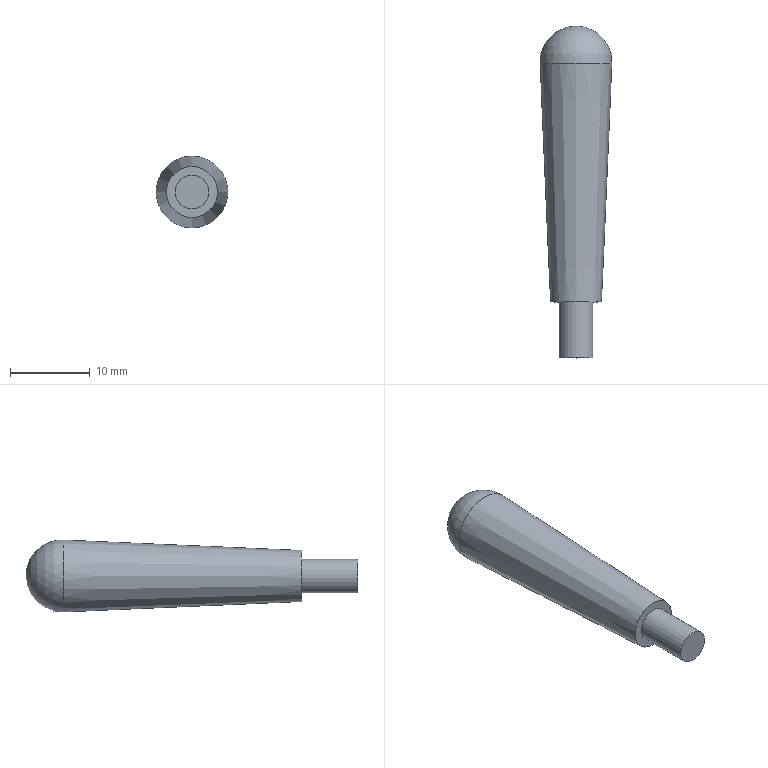Component | NX | HANDLE | 1 solid | 5 faces | box 9 x 41.5 x 9 mm | volume 1698 mm3 | plane 2 | sphere 1 | cone 1 | cylinder 1 | commonest cylinder face diameters 4.2 x1
STEP:
#1=CARTESIAN_POINT('',(0.,0.,0.));
#2=DIRECTION('',(0.,0.,1.));
#3=DIRECTION('',(1.,0.,0.));
#4=AXIS2_PLACEMENT_3D('',#1,#2,#3);
#5=CARTESIAN_POINT('',(0.,69.,123.5));
#6=VERTEX_POINT('',#5);
#7=CARTESIAN_POINT('',(0.,69.,125.6));
#8=DIRECTION('',(0.,-1.,0.));
#9=DIRECTION('',(0.,0.,-1.));
#10=AXIS2_PLACEMENT_3D('',#7,#8,#9);
#11=CIRCLE('',#10,2.1);
#12=CARTESIAN_POINT('',(0.,69.,127.7));
#13=DIRECTION('',(0.,1.,0.));
#14=DIRECTION('',(0.,0.,1.));
#15=AXIS2_PLACEMENT_3D('',#12,#13,#14);
#16=PLANE('',#15);
#17=CARTESIAN_POINT('',(-4.2,0.));
#18=CARTESIAN_POINT('',(-4.2,3.637));
#19=CARTESIAN_POINT('',(-1.05,1.819));
#20=CARTESIAN_POINT('',(2.1,0.));
#21=CARTESIAN_POINT('',(-1.05,-1.819));
#22=CARTESIAN_POINT('',(-4.2,-3.637));
#23=CARTESIAN_POINT('',(-4.2,0.));
#24=(BOUNDED_CURVE()B_SPLINE_CURVE(2,(#17,#18,#19,#20,#21,#22,#23),.UNSPECIFIED.,.T.,.F.)B_SPLINE_CURVE_WITH_KNOTS((1,2,2,2,2,1),(-2.094,0.,2.094,4.189,6.283,8.378),.UNSPECIFIED.)CURVE()GEOMETRIC_REPRESENTATION_ITEM()RATIONAL_B_SPLINE_CURVE((1.,0.5,1.,0.5,1.,0.5,1.))REPRESENTATION_ITEM(''));
#25=(GEOMETRIC_REPRESENTATION_CONTEXT(2)PARAMETRIC_REPRESENTATION_CONTEXT()REPRESENTATION_CONTEXT('',''));
#26=DEFINITIONAL_REPRESENTATION('',(#24),#25);
#27=PCURVE('',#16,#26);
#28=CARTESIAN_POINT('',(0.,69.,125.6));
#29=DIRECTION('',(0.,-1.,0.));
#30=DIRECTION('',(0.,0.,-1.));
#31=AXIS2_PLACEMENT_3D('',#28,#29,#30);
#32=CYLINDRICAL_SURFACE('',#31,2.1);
#33=CARTESIAN_POINT('',(0.,0.));
#34=DIRECTION('',(1.,0.));
#35=VECTOR('',#34,1.);
#36=LINE('',#33,#35);
#37=(GEOMETRIC_REPRESENTATION_CONTEXT(2)PARAMETRIC_REPRESENTATION_CONTEXT()REPRESENTATION_CONTEXT('',''));
#38=DEFINITIONAL_REPRESENTATION('',(#36),#37);
#39=PCURVE('',#32,#38);
#40=SURFACE_CURVE('',#11,(#27,#39),.PCURVE_S1.);
#41=EDGE_CURVE('',#6,#6,#40,.T.);
#42=ORIENTED_EDGE('',*,*,#41,.T.);
#43=EDGE_LOOP('',(#42));
#44=FACE_BOUND('',#43,.T.);
#45=ADVANCED_FACE('',(#44),#16,.F.);
#46=CARTESIAN_POINT('',(-0.,105.804,130.096));
#47=VERTEX_POINT('',#46);
#48=CARTESIAN_POINT('',(0.,105.804,121.104));
#49=VERTEX_POINT('',#48);
#50=CARTESIAN_POINT('',(0.,105.804,125.6));
#51=DIRECTION('',(0.,-1.,0.));
#52=DIRECTION('',(0.,0.,-1.));
#53=AXIS2_PLACEMENT_3D('',#50,#51,#52);
#54=CIRCLE('',#53,4.496);
#55=CARTESIAN_POINT('',(0.,106.,125.6));
#56=DIRECTION('',(0.,-1.,0.));
#57=DIRECTION('',(0.,0.,1.));
#58=AXIS2_PLACEMENT_3D('',#55,#56,#57);
#59=SPHERICAL_SURFACE('',#58,4.5);
#60=CARTESIAN_POINT('',(-3.142,0.04363));
#61=CARTESIAN_POINT('',(-3.046,0.04363));
#62=CARTESIAN_POINT('',(-2.856,0.04363));
#63=CARTESIAN_POINT('',(-2.57,0.04363));
#64=CARTESIAN_POINT('',(-2.285,0.04363));
#65=CARTESIAN_POINT('',(-1.999,0.04363));
#66=CARTESIAN_POINT('',(-1.714,0.04363));
#67=CARTESIAN_POINT('',(-1.428,0.04363));
#68=CARTESIAN_POINT('',(-1.142,0.04363));
#69=CARTESIAN_POINT('',(-0.8568,0.04363));
#70=CARTESIAN_POINT('',(-0.5712,0.04363));
#71=CARTESIAN_POINT('',(-0.2856,0.04363));
#72=CARTESIAN_POINT('',(0.,0.04363));
#73=CARTESIAN_POINT('',(0.2856,0.04363));
#74=CARTESIAN_POINT('',(0.5712,0.04363));
#75=CARTESIAN_POINT('',(0.8568,0.04363));
#76=CARTESIAN_POINT('',(1.142,0.04363));
#77=CARTESIAN_POINT('',(1.428,0.04363));
#78=CARTESIAN_POINT('',(1.714,0.04363));
#79=CARTESIAN_POINT('',(1.999,0.04363));
#80=CARTESIAN_POINT('',(2.285,0.04363));
#81=CARTESIAN_POINT('',(2.57,0.04363));
#82=CARTESIAN_POINT('',(2.856,0.04363));
#83=CARTESIAN_POINT('',(3.046,0.04363));
#84=CARTESIAN_POINT('',(3.142,0.04363));
#85=B_SPLINE_CURVE_WITH_KNOTS('',3,(#60,#61,#62,#63,#64,#65,#66,#67,#68,#69,#70,#71,#72,#73,#74,#75,#76,#77,#78,#79,#80,#81,#82,#83,#84),.UNSPECIFIED.,.F.,.F.,(4,1,1,1,1,1,1,1,1,1,1,1,1,1,1,1,1,1,1,1,1,1,4),(0.,0.2856,0.5712,0.8568,1.142,1.428,1.714,1.999,2.285,2.57,2.856,3.142,3.427,3.713,3.998,4.284,4.57,4.855,5.141,5.426,5.712,5.998,6.283),.QUASI_UNIFORM_KNOTS.);
#86=(GEOMETRIC_REPRESENTATION_CONTEXT(2)PARAMETRIC_REPRESENTATION_CONTEXT()REPRESENTATION_CONTEXT('',''));
#87=DEFINITIONAL_REPRESENTATION('',(#85),#86);
#88=PCURVE('',#59,#87);
#89=CARTESIAN_POINT('',(0.,105.804,125.6));
#90=DIRECTION('',(0.,1.,0.));
#91=DIRECTION('',(0.,0.,1.));
#92=AXIS2_PLACEMENT_3D('',#89,#90,#91);
#93=CONICAL_SURFACE('',#92,4.496,0.04363);
#94=CARTESIAN_POINT('',(9.425,0.));
#95=DIRECTION('',(-1.,0.));
#96=VECTOR('',#95,1.);
#97=LINE('',#94,#96);
#98=(GEOMETRIC_REPRESENTATION_CONTEXT(2)PARAMETRIC_REPRESENTATION_CONTEXT()REPRESENTATION_CONTEXT('',''));
#99=DEFINITIONAL_REPRESENTATION('',(#97),#98);
#100=PCURVE('',#93,#99);
#101=SURFACE_CURVE('',#54,(#88,#100),.PCURVE_S1.);
#102=EDGE_CURVE('',#47,#49,#101,.T.);
#103=ORIENTED_EDGE('',*,*,#102,.F.);
#104=CARTESIAN_POINT('',(0.,110.5,125.6));
#105=VERTEX_POINT('',#104);
#106=CARTESIAN_POINT('',(-0.,110.5,125.6));
#107=CARTESIAN_POINT('',(0.,110.5,126.811));
#108=CARTESIAN_POINT('',(0.,110.109,128.022));
#109=CARTESIAN_POINT('',(0.,109.327,129.075));
#110=CARTESIAN_POINT('',(0.,108.24,129.811));
#111=CARTESIAN_POINT('',(0.,107.013,130.149));
#112=CARTESIAN_POINT('',(0.,105.804,130.096));
#113=B_SPLINE_CURVE_WITH_KNOTS('',6,(#106,#107,#108,#109,#110,#111,#112),.UNSPECIFIED.,.F.,.F.,(7,7),(-1.571,0.04363),.PIECEWISE_BEZIER_KNOTS.);
#114=CARTESIAN_POINT('',(0.,0.));
#115=DIRECTION('',(0.,1.));
#116=VECTOR('',#115,1.);
#117=LINE('',#114,#116);
#118=(GEOMETRIC_REPRESENTATION_CONTEXT(2)PARAMETRIC_REPRESENTATION_CONTEXT()REPRESENTATION_CONTEXT('',''));
#119=DEFINITIONAL_REPRESENTATION('',(#117),#118);
#120=PCURVE('',#59,#119);
#121=CARTESIAN_POINT('',(6.283,0.));
#122=DIRECTION('',(0.,1.));
#123=VECTOR('',#122,1.);
#124=LINE('',#121,#123);
#125=(GEOMETRIC_REPRESENTATION_CONTEXT(2)PARAMETRIC_REPRESENTATION_CONTEXT()REPRESENTATION_CONTEXT('',''));
#126=DEFINITIONAL_REPRESENTATION('',(#124),#125);
#127=PCURVE('',#59,#126);
#128=SEAM_CURVE('',#113,(#120,#127),.PCURVE_S1.);
#129=EDGE_CURVE('',#105,#47,#128,.T.);
#130=ORIENTED_EDGE('',*,*,#129,.F.);
#131=ORIENTED_EDGE('',*,*,#129,.T.);
#132=CARTESIAN_POINT('',(0.,105.804,125.6));
#133=DIRECTION('',(0.,-1.,0.));
#134=DIRECTION('',(0.,0.,-1.));
#135=AXIS2_PLACEMENT_3D('',#132,#133,#134);
#136=CIRCLE('',#135,4.496);
#137=CARTESIAN_POINT('',(3.142,0.04363));
#138=CARTESIAN_POINT('',(3.237,0.04363));
#139=CARTESIAN_POINT('',(3.427,0.04363));
#140=CARTESIAN_POINT('',(3.713,0.04363));
#141=CARTESIAN_POINT('',(3.998,0.04363));
#142=CARTESIAN_POINT('',(4.284,0.04363));
#143=CARTESIAN_POINT('',(4.57,0.04363));
#144=CARTESIAN_POINT('',(4.855,0.04363));
#145=CARTESIAN_POINT('',(5.141,0.04363));
#146=CARTESIAN_POINT('',(5.426,0.04363));
#147=CARTESIAN_POINT('',(5.712,0.04363));
#148=CARTESIAN_POINT('',(5.998,0.04363));
#149=CARTESIAN_POINT('',(6.283,0.04363));
#150=CARTESIAN_POINT('',(6.569,0.04363));
#151=CARTESIAN_POINT('',(6.854,0.04363));
#152=CARTESIAN_POINT('',(7.14,0.04363));
#153=CARTESIAN_POINT('',(7.426,0.04363));
#154=CARTESIAN_POINT('',(7.711,0.04363));
#155=CARTESIAN_POINT('',(7.997,0.04363));
#156=CARTESIAN_POINT('',(8.282,0.04363));
#157=CARTESIAN_POINT('',(8.568,0.04363));
#158=CARTESIAN_POINT('',(8.854,0.04363));
#159=CARTESIAN_POINT('',(9.139,0.04363));
#160=CARTESIAN_POINT('',(9.33,0.04363));
#161=CARTESIAN_POINT('',(9.425,0.04363));
#162=B_SPLINE_CURVE_WITH_KNOTS('',3,(#137,#138,#139,#140,#141,#142,#143,#144,#145,#146,#147,#148,#149,#150,#151,#152,#153,#154,#155,#156,#157,#158,#159,#160,#161),.UNSPECIFIED.,.F.,.F.,(4,1,1,1,1,1,1,1,1,1,1,1,1,1,1,1,1,1,1,1,1,1,4),(0.,0.2856,0.5712,0.8568,1.142,1.428,1.714,1.999,2.285,2.57,2.856,3.142,3.427,3.713,3.998,4.284,4.57,4.855,5.141,5.426,5.712,5.998,6.283),.QUASI_UNIFORM_KNOTS.);
#163=(GEOMETRIC_REPRESENTATION_CONTEXT(2)PARAMETRIC_REPRESENTATION_CONTEXT()REPRESENTATION_CONTEXT('',''));
#164=DEFINITIONAL_REPRESENTATION('',(#162),#163);
#165=PCURVE('',#59,#164);
#166=CARTESIAN_POINT('',(9.425,0.));
#167=DIRECTION('',(-1.,0.));
#168=VECTOR('',#167,1.);
#169=LINE('',#166,#168);
#170=(GEOMETRIC_REPRESENTATION_CONTEXT(2)PARAMETRIC_REPRESENTATION_CONTEXT()REPRESENTATION_CONTEXT('',''));
#171=DEFINITIONAL_REPRESENTATION('',(#169),#170);
#172=PCURVE('',#93,#171);
#173=SURFACE_CURVE('',#136,(#165,#172),.PCURVE_S1.);
#174=EDGE_CURVE('',#49,#47,#173,.T.);
#175=ORIENTED_EDGE('',*,*,#174,.F.);
#176=EDGE_LOOP('',(#103,#130,#131,#175));
#177=FACE_BOUND('',#176,.T.);
#178=ADVANCED_FACE('',(#177),#59,.T.);
#179=CARTESIAN_POINT('',(0.,76.,122.406));
#180=VERTEX_POINT('',#179);
#181=CARTESIAN_POINT('',(0.,76.,125.6));
#182=DIRECTION('',(0.,-1.,0.));
#183=DIRECTION('',(0.,0.,-1.));
#184=AXIS2_PLACEMENT_3D('',#181,#182,#183);
#185=CIRCLE('',#184,3.194);
#186=CARTESIAN_POINT('',(9.425,-29.804));
#187=DIRECTION('',(-1.,0.));
#188=VECTOR('',#187,1.);
#189=LINE('',#186,#188);
#190=(GEOMETRIC_REPRESENTATION_CONTEXT(2)PARAMETRIC_REPRESENTATION_CONTEXT()REPRESENTATION_CONTEXT('',''));
#191=DEFINITIONAL_REPRESENTATION('',(#189),#190);
#192=PCURVE('',#93,#191);
#193=CARTESIAN_POINT('',(0.,76.,128.794));
#194=DIRECTION('',(0.,1.,0.));
#195=DIRECTION('',(0.,0.,1.));
#196=AXIS2_PLACEMENT_3D('',#193,#194,#195);
#197=PLANE('',#196);
#198=CARTESIAN_POINT('',(-6.389,0.));
#199=CARTESIAN_POINT('',(-6.389,5.533));
#200=CARTESIAN_POINT('',(-1.597,2.766));
#201=CARTESIAN_POINT('',(3.194,0.));
#202=CARTESIAN_POINT('',(-1.597,-2.766));
#203=CARTESIAN_POINT('',(-6.389,-5.533));
#204=CARTESIAN_POINT('',(-6.389,0.));
#205=(BOUNDED_CURVE()B_SPLINE_CURVE(2,(#198,#199,#200,#201,#202,#203,#204),.UNSPECIFIED.,.T.,.F.)B_SPLINE_CURVE_WITH_KNOTS((1,2,2,2,2,1),(-2.094,0.,2.094,4.189,6.283,8.378),.UNSPECIFIED.)CURVE()GEOMETRIC_REPRESENTATION_ITEM()RATIONAL_B_SPLINE_CURVE((1.,0.5,1.,0.5,1.,0.5,1.))REPRESENTATION_ITEM(''));
#206=(GEOMETRIC_REPRESENTATION_CONTEXT(2)PARAMETRIC_REPRESENTATION_CONTEXT()REPRESENTATION_CONTEXT('',''));
#207=DEFINITIONAL_REPRESENTATION('',(#205),#206);
#208=PCURVE('',#197,#207);
#209=SURFACE_CURVE('',#185,(#192,#208),.PCURVE_S1.);
#210=EDGE_CURVE('',#180,#180,#209,.T.);
#211=ORIENTED_EDGE('',*,*,#210,.F.);
#212=CARTESIAN_POINT('',(0.,76.,122.406));
#213=CARTESIAN_POINT('',(0.,105.804,121.104));
#214=B_SPLINE_CURVE_WITH_KNOTS('',1,(#212,#213),.UNSPECIFIED.,.F.,.F.,(2,2),(-29.832,0.),.PIECEWISE_BEZIER_KNOTS.);
#215=CARTESIAN_POINT('',(9.425,0.));
#216=DIRECTION('',(0.,1.));
#217=VECTOR('',#216,1.);
#218=LINE('',#215,#217);
#219=(GEOMETRIC_REPRESENTATION_CONTEXT(2)PARAMETRIC_REPRESENTATION_CONTEXT()REPRESENTATION_CONTEXT('',''));
#220=DEFINITIONAL_REPRESENTATION('',(#218),#219);
#221=PCURVE('',#93,#220);
#222=CARTESIAN_POINT('',(3.142,0.));
#223=DIRECTION('',(0.,1.));
#224=VECTOR('',#223,1.);
#225=LINE('',#222,#224);
#226=(GEOMETRIC_REPRESENTATION_CONTEXT(2)PARAMETRIC_REPRESENTATION_CONTEXT()REPRESENTATION_CONTEXT('',''));
#227=DEFINITIONAL_REPRESENTATION('',(#225),#226);
#228=PCURVE('',#93,#227);
#229=SEAM_CURVE('',#214,(#221,#228),.PCURVE_S1.);
#230=EDGE_CURVE('',#180,#49,#229,.T.);
#231=ORIENTED_EDGE('',*,*,#230,.T.);
#232=ORIENTED_EDGE('',*,*,#174,.T.);
#233=ORIENTED_EDGE('',*,*,#102,.T.);
#234=ORIENTED_EDGE('',*,*,#230,.F.);
#235=EDGE_LOOP('',(#211,#231,#232,#233,#234));
#236=FACE_BOUND('',#235,.T.);
#237=ADVANCED_FACE('',(#236),#93,.T.);
#238=CARTESIAN_POINT('',(0.,76.,123.5));
#239=VERTEX_POINT('',#238);
#240=CARTESIAN_POINT('',(0.,76.,125.6));
#241=DIRECTION('',(0.,-1.,0.));
#242=DIRECTION('',(0.,0.,-1.));
#243=AXIS2_PLACEMENT_3D('',#240,#241,#242);
#244=CIRCLE('',#243,2.1);
#245=CARTESIAN_POINT('',(-5.294,0.));
#246=CARTESIAN_POINT('',(-5.294,3.637));
#247=CARTESIAN_POINT('',(-2.144,1.819));
#248=CARTESIAN_POINT('',(1.006,0.));
#249=CARTESIAN_POINT('',(-2.144,-1.819));
#250=CARTESIAN_POINT('',(-5.294,-3.637));
#251=CARTESIAN_POINT('',(-5.294,0.));
#252=(BOUNDED_CURVE()B_SPLINE_CURVE(2,(#245,#246,#247,#248,#249,#250,#251),.UNSPECIFIED.,.T.,.F.)B_SPLINE_CURVE_WITH_KNOTS((1,2,2,2,2,1),(-2.094,0.,2.094,4.189,6.283,8.378),.UNSPECIFIED.)CURVE()GEOMETRIC_REPRESENTATION_ITEM()RATIONAL_B_SPLINE_CURVE((1.,0.5,1.,0.5,1.,0.5,1.))REPRESENTATION_ITEM(''));
#253=(GEOMETRIC_REPRESENTATION_CONTEXT(2)PARAMETRIC_REPRESENTATION_CONTEXT()REPRESENTATION_CONTEXT('',''));
#254=DEFINITIONAL_REPRESENTATION('',(#252),#253);
#255=PCURVE('',#197,#254);
#256=CARTESIAN_POINT('',(0.,-7.));
#257=DIRECTION('',(1.,0.));
#258=VECTOR('',#257,1.);
#259=LINE('',#256,#258);
#260=(GEOMETRIC_REPRESENTATION_CONTEXT(2)PARAMETRIC_REPRESENTATION_CONTEXT()REPRESENTATION_CONTEXT('',''));
#261=DEFINITIONAL_REPRESENTATION('',(#259),#260);
#262=PCURVE('',#32,#261);
#263=SURFACE_CURVE('',#244,(#255,#262),.PCURVE_S1.);
#264=EDGE_CURVE('',#239,#239,#263,.T.);
#265=ORIENTED_EDGE('',*,*,#264,.F.);
#266=EDGE_LOOP('',(#265));
#267=FACE_BOUND('',#266,.T.);
#268=ORIENTED_EDGE('',*,*,#210,.T.);
#269=EDGE_LOOP('',(#268));
#270=FACE_BOUND('',#269,.T.);
#271=ADVANCED_FACE('',(#267,#270),#197,.F.);
#272=ORIENTED_EDGE('',*,*,#41,.F.);
#273=CARTESIAN_POINT('',(-0.,76.,123.5));
#274=CARTESIAN_POINT('',(-0.,69.,123.5));
#275=B_SPLINE_CURVE_WITH_KNOTS('',1,(#273,#274),.UNSPECIFIED.,.F.,.F.,(2,2),(-7.,0.),.PIECEWISE_BEZIER_KNOTS.);
#276=CARTESIAN_POINT('',(0.,0.));
#277=DIRECTION('',(0.,1.));
#278=VECTOR('',#277,1.);
#279=LINE('',#276,#278);
#280=(GEOMETRIC_REPRESENTATION_CONTEXT(2)PARAMETRIC_REPRESENTATION_CONTEXT()REPRESENTATION_CONTEXT('',''));
#281=DEFINITIONAL_REPRESENTATION('',(#279),#280);
#282=PCURVE('',#32,#281);
#283=CARTESIAN_POINT('',(6.283,0.));
#284=DIRECTION('',(0.,1.));
#285=VECTOR('',#284,1.);
#286=LINE('',#283,#285);
#287=(GEOMETRIC_REPRESENTATION_CONTEXT(2)PARAMETRIC_REPRESENTATION_CONTEXT()REPRESENTATION_CONTEXT('',''));
#288=DEFINITIONAL_REPRESENTATION('',(#286),#287);
#289=PCURVE('',#32,#288);
#290=SEAM_CURVE('',#275,(#282,#289),.PCURVE_S1.);
#291=EDGE_CURVE('',#239,#6,#290,.T.);
#292=ORIENTED_EDGE('',*,*,#291,.F.);
#293=ORIENTED_EDGE('',*,*,#264,.T.);
#294=ORIENTED_EDGE('',*,*,#291,.T.);
#295=EDGE_LOOP('',(#272,#292,#293,#294));
#296=FACE_BOUND('',#295,.T.);
#297=ADVANCED_FACE('',(#296),#32,.T.);
#298=CLOSED_SHELL('',(#45,#178,#237,#271,#297));
#299=MANIFOLD_SOLID_BREP('',#298);
#300=(LENGTH_UNIT()NAMED_UNIT(*)SI_UNIT(.MILLI.,.METRE.));
#301=UNCERTAINTY_MEASURE_WITH_UNIT(LENGTH_MEASURE(0.00001),#300,'','');
#302=(NAMED_UNIT(*)PLANE_ANGLE_UNIT()SI_UNIT($,.RADIAN.));
#303=(NAMED_UNIT(*)SI_UNIT($,.STERADIAN.)SOLID_ANGLE_UNIT());
#304=(GEOMETRIC_REPRESENTATION_CONTEXT(3)GLOBAL_UNCERTAINTY_ASSIGNED_CONTEXT((#301))GLOBAL_UNIT_ASSIGNED_CONTEXT((#300,#302,#303))REPRESENTATION_CONTEXT('',''));
#305=ADVANCED_BREP_SHAPE_REPRESENTATION('',(#4,#299),#304);